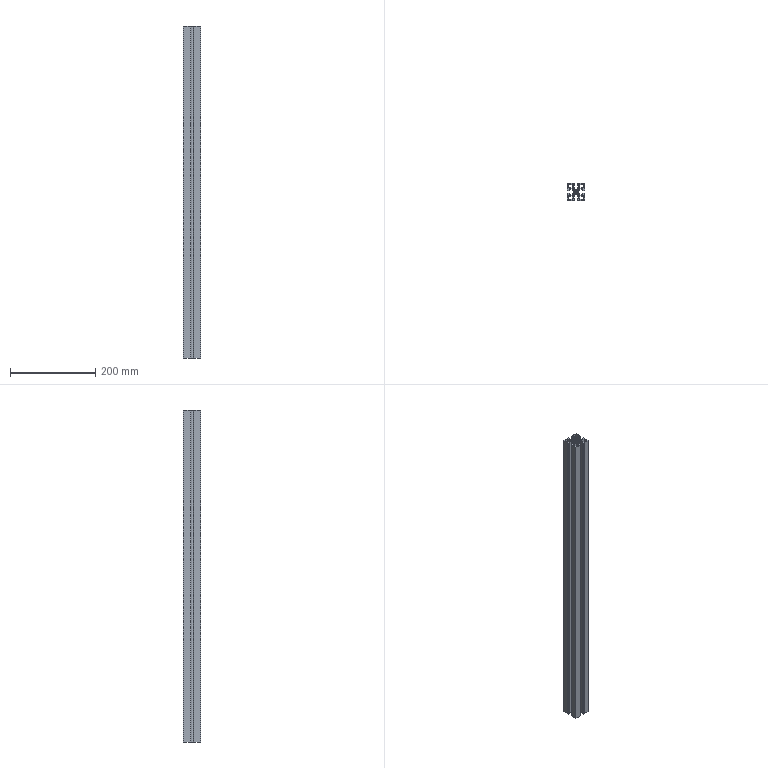Component | SolidWorks | AluminumProfile780-2 | 1 solid | 89 faces | box 40 x 40 x 780 mm | volume 452458 mm3 | plane 82 | cylinder 7 | commonest cylinder face diameters 10.5 x5 6.8 x2 | material 6061 Alloy
build123d program:
from build123d import *

# Parameters (mm, degrees)
SKETCH1_W                  = 40
SKETCH1_H                  = 40
EXTRUDE1_DEPTH             = 1640
CUT_EXTRUDE1_DEPTH         = 1641.975
SKETCH3_R                  = 3.4
CUT_EXTRUDE2_DEPTH         = 1641.975
CIRPATTERN1_COUNT          = 4
EXTRUDE2_DEPTH             = 1641.975
CIRPATTERN2_COUNT          = 4
SKETCH5_W                  = 9
SKETCH5_H                  = 9
EXTRUDE3_DEPTH             = 1641.975
CIRPATTERN3_COUNT          = 4
M8X1_25_TAPPED_HOLE3_D     = 6.8
M8X1_25_TAPPED_HOLE3_DEPTH = 19.75
M8X1_25_TAPPED_HOLE3_TIP   = 2.043
SKETCH9_W                  = 177.591
SKETCH9_H                  = 2021.808
CUT_EXTRUDE3_DEPTH         = 1641.975


with BuildPart() as part:
    # Sketch1 → Extrude1 (new body)
    with BuildSketch(Plane.XY):
        with Locations((20, 20)):
            Rectangle(SKETCH1_W, SKETCH1_H)
    extrude(amount=EXTRUDE1_DEPTH)

    # Sketch2 → Cut-Extrude1 (cut, through all)
    with BuildSketch(Plane.XY.offset(1640)):
        Polygon((16, 40), (16, 36), (13, 36), (13, 29), (27, 29), (27, 36), (24, 36), (24, 40), align=None)
    cut_extrude1 = extrude(amount=-CUT_EXTRUDE1_DEPTH, mode=Mode.SUBTRACT)

    # Sketch3 → Cut-Extrude2 (cut, through all)
    with BuildSketch(Plane.XY.offset(1640)):
        with Locations((20, 20)):
            Circle(SKETCH3_R)
    extrude(amount=-CUT_EXTRUDE2_DEPTH, mode=Mode.SUBTRACT)

    # CirPattern1: Cut-Extrude1 ×4 about axis
    cirpattern1_axis = Axis((20, 20, 0), (0, 0, 1))
    for i in range(1, CIRPATTERN1_COUNT):
        add(cut_extrude1.rotate(cirpattern1_axis, i * 360 / CIRPATTERN1_COUNT), mode=Mode.SUBTRACT)

    # Sketch4 → Extrude2 (cut, through all)
    with BuildSketch(Plane.XY.offset(1640)):
        with BuildLine():
            Line((15.75, 29), (16.457, 28.293))
            Line((16.457, 28.293), (14.806, 26.641))
            Line((14.806, 26.641), (17.082, 24.365))
            ThreePointArc((17.082, 24.365), (20, 25.25), (22.918, 24.365))
            Line((22.918, 24.365), (25.194, 26.641))
            Line((25.194, 26.641), (23.543, 28.293))
            Line((23.543, 28.293), (24.25, 29))
            Line((24.25, 29), (15.75, 29))
        make_face()
    extrude2 = extrude(amount=-EXTRUDE2_DEPTH, mode=Mode.SUBTRACT)

    # CirPattern2: Extrude2 ×4 about axis
    cirpattern2_axis = Axis((20, 20, 0), (0, 0, 1))
    for i in range(1, CIRPATTERN2_COUNT):
        add(extrude2.rotate(cirpattern2_axis, i * 360 / CIRPATTERN2_COUNT), mode=Mode.SUBTRACT)

    # Sketch5 → Extrude3 (cut, through all)
    with BuildSketch(Plane.XY.offset(1640)):
        with Locations((6.5, 33.5)):
            Rectangle(SKETCH5_W, SKETCH5_H)
    extrude3 = extrude(amount=-EXTRUDE3_DEPTH, mode=Mode.SUBTRACT)

    # CirPattern3: Extrude3 ×4 about axis
    cirpattern3_axis = Axis((20, 20, 0), (0, 0, 1))
    for i in range(1, CIRPATTERN3_COUNT):
        add(extrude3.rotate(cirpattern3_axis, i * 360 / CIRPATTERN3_COUNT), mode=Mode.SUBTRACT)

    # M8x1.25 Tapped Hole3
    with Locations(Plane(origin=(20, 20, 1640), x_dir=(1, 0, 0), z_dir=(0, 0, 1))):
        with Locations((0, 0)):
            Hole(M8X1_25_TAPPED_HOLE3_D / 2, depth=M8X1_25_TAPPED_HOLE3_DEPTH)
            with Locations((0, 0, -(M8X1_25_TAPPED_HOLE3_DEPTH + M8X1_25_TAPPED_HOLE3_TIP / 2))):  # 118° drill point
                Cone(0, M8X1_25_TAPPED_HOLE3_D / 2, M8X1_25_TAPPED_HOLE3_TIP, mode=Mode.SUBTRACT)

    # Sketch9 → Cut-Extrude3 (cut, through all)
    with BuildSketch(Plane.XZ):
        with Locations((13.869, 1790.904)):
            Rectangle(SKETCH9_W, SKETCH9_H)
    extrude(amount=-CUT_EXTRUDE3_DEPTH, mode=Mode.SUBTRACT)


solid = part.part

# Placed as in the assembly
solid = solid.moved(Location((-768.352, -1008.217, -96.285), (0, 0, 0)))